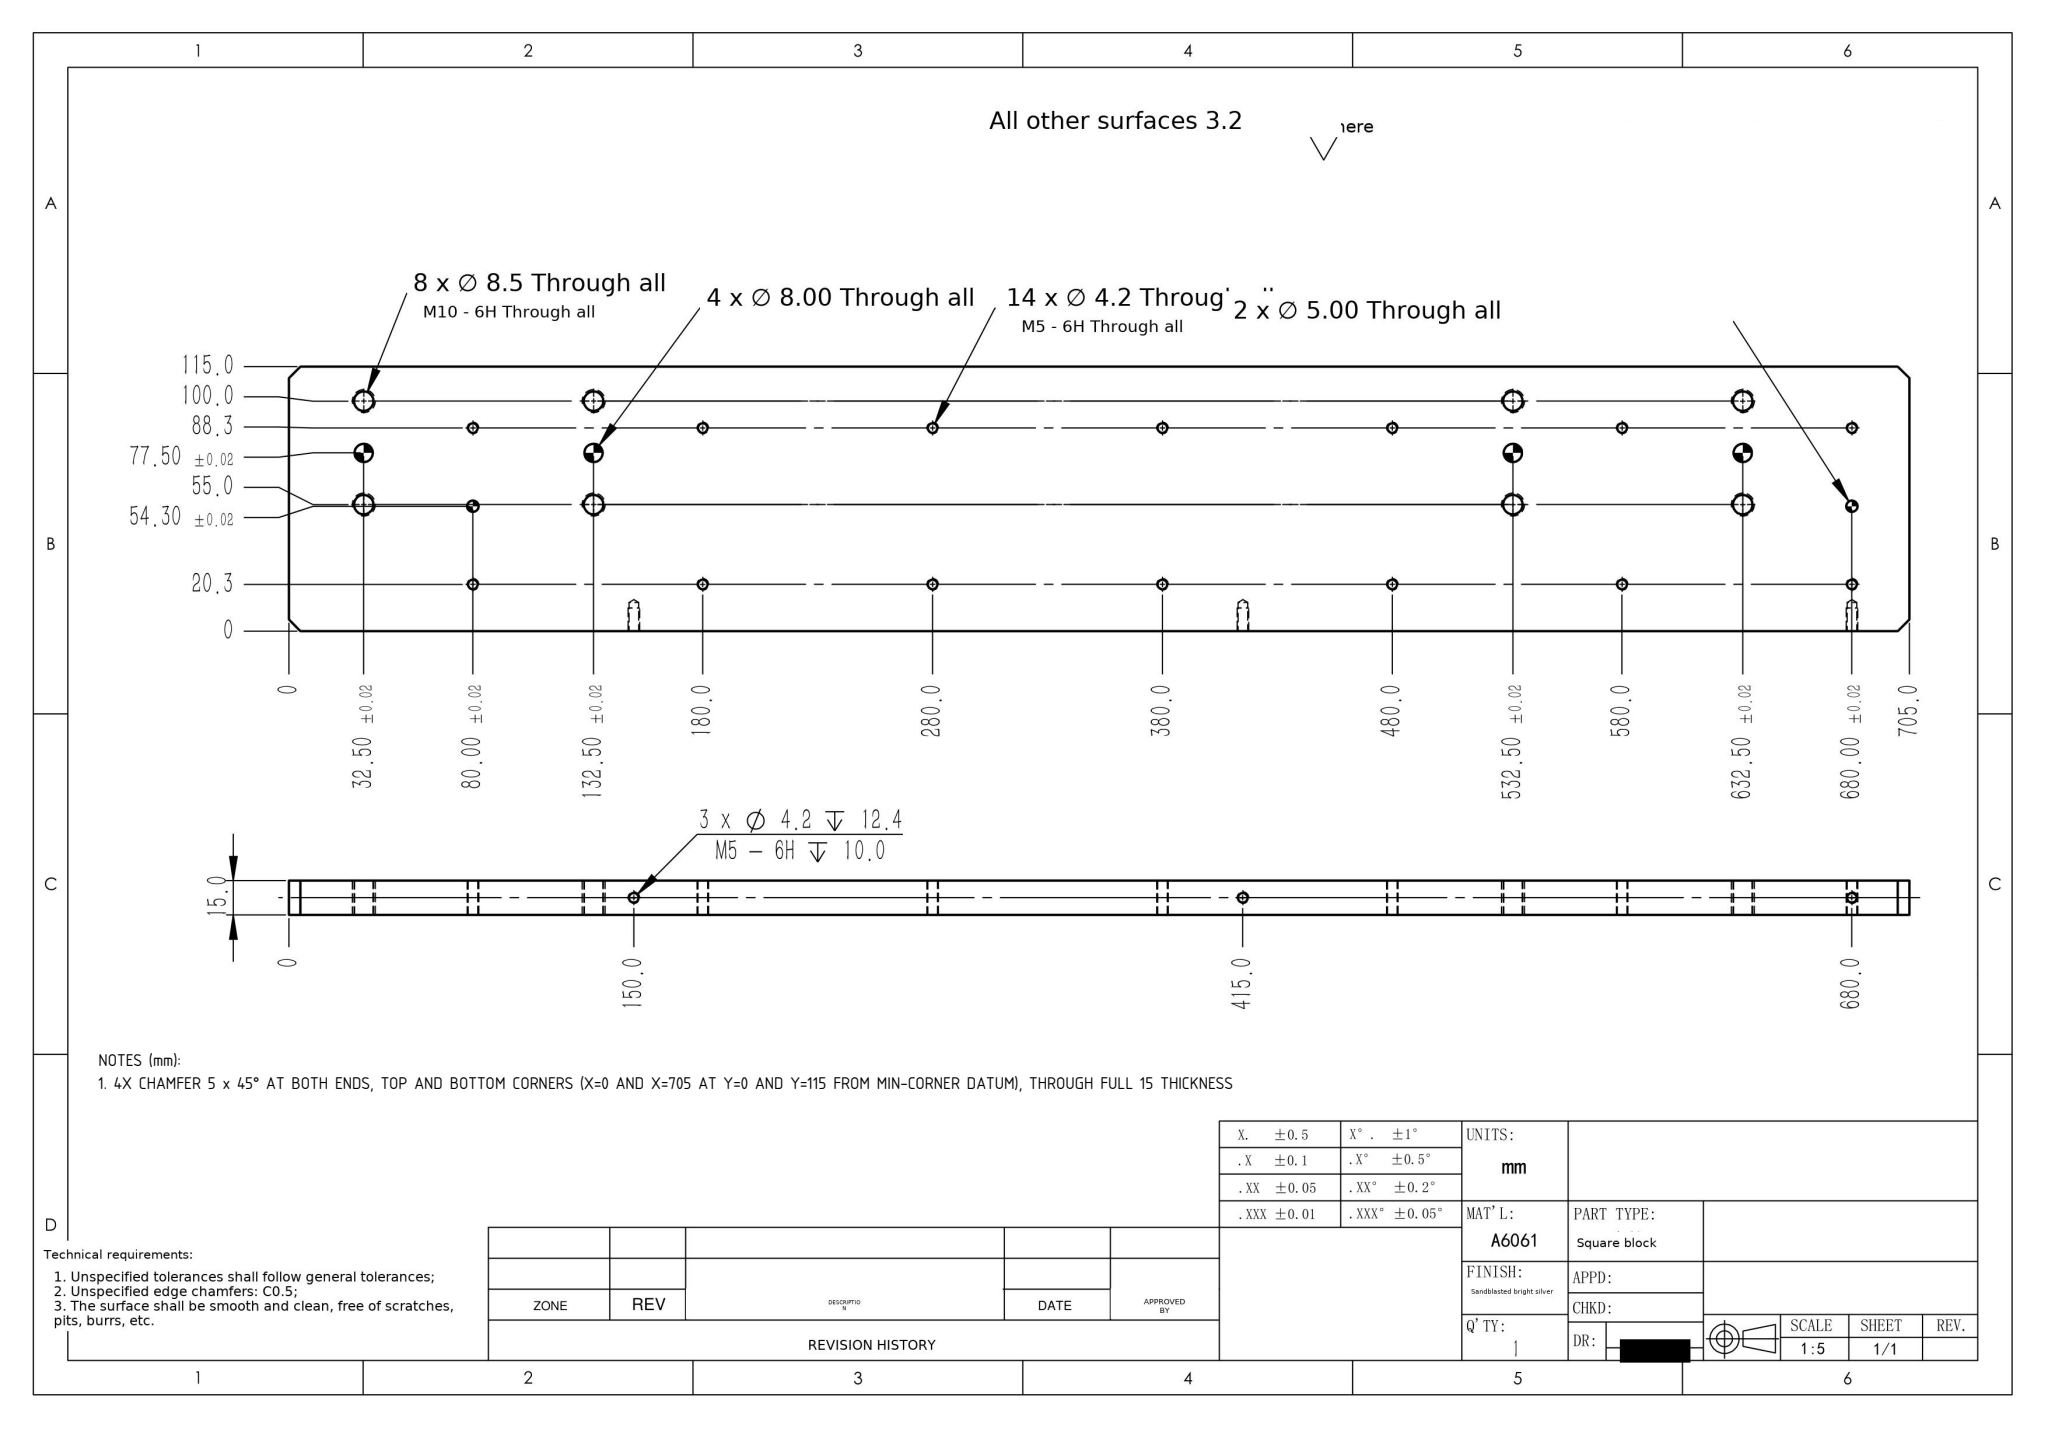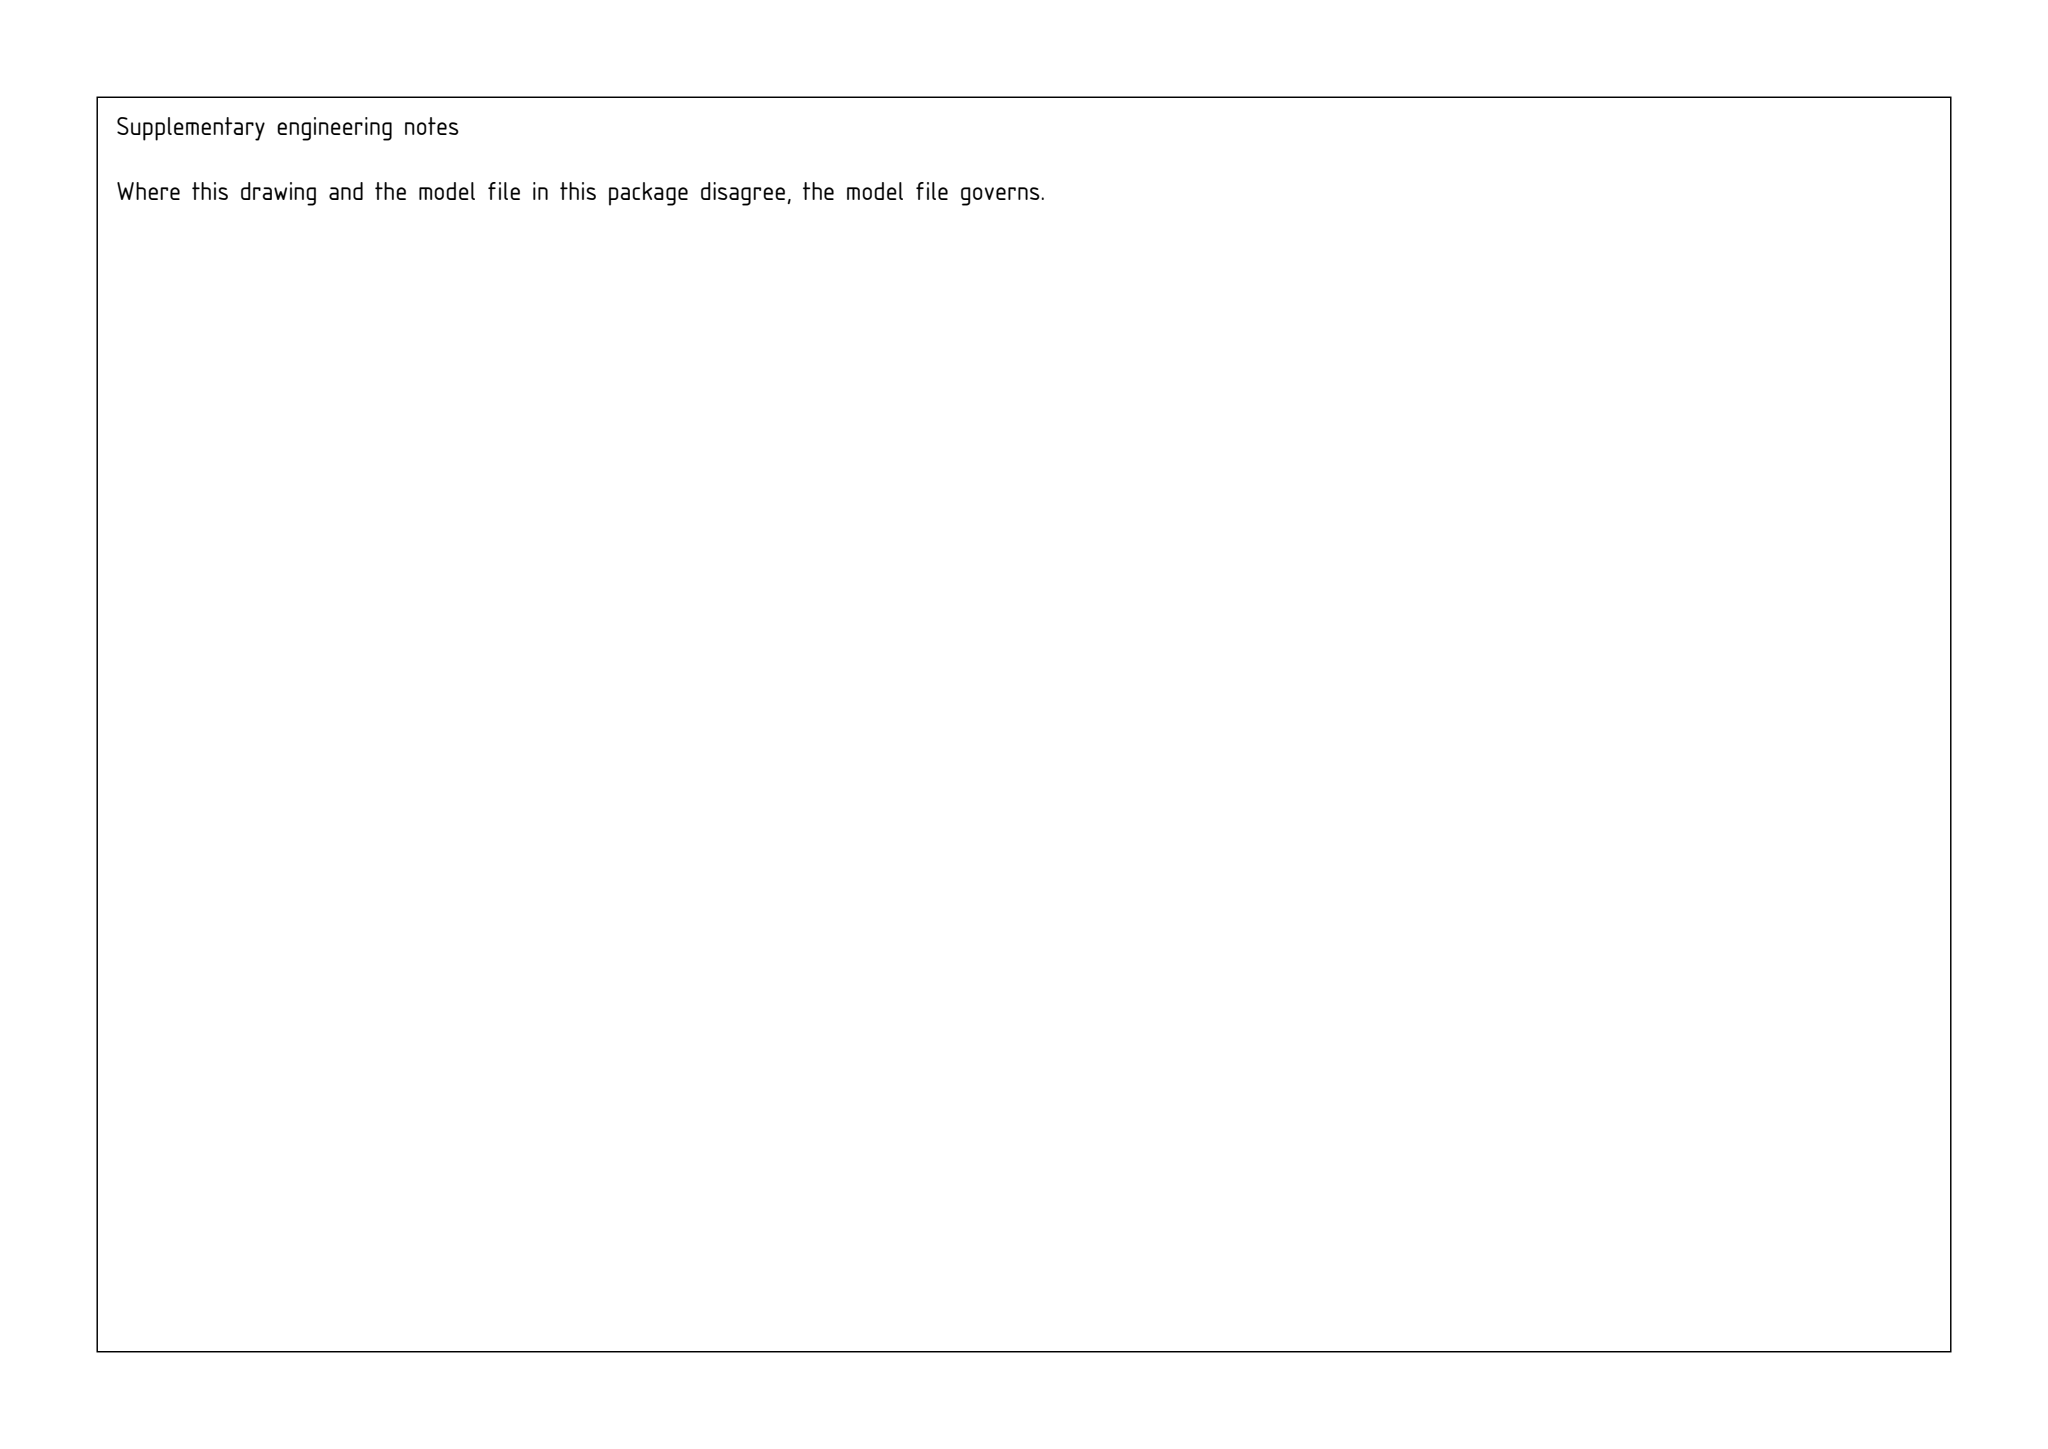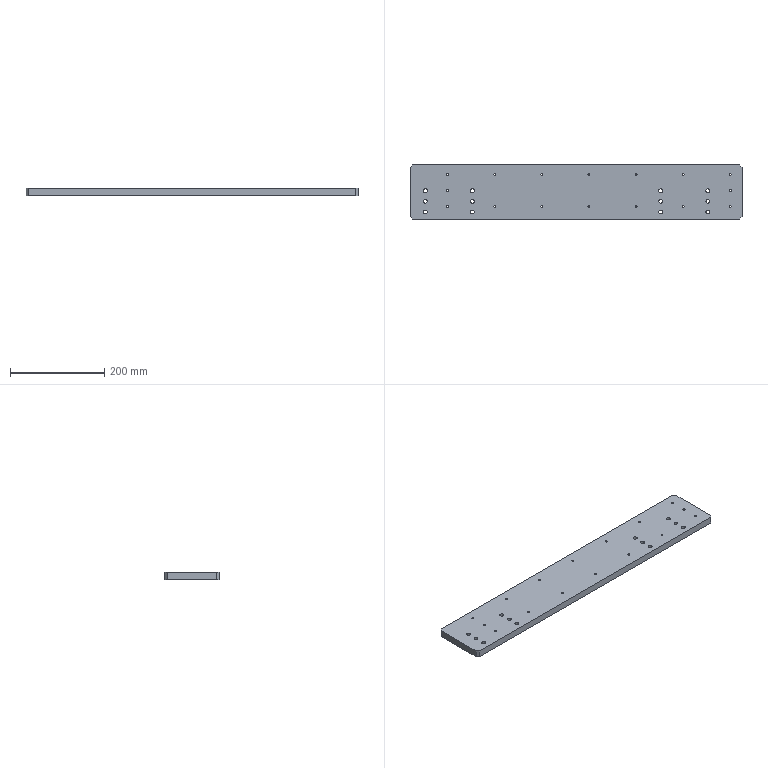Part | SolidWorks | mm | 1 solid | 78 faces | box 705 x 115 x 15 mm | volume 1201518 mm3 | cylinder 62 | plane 10 | cone 6 | commonest cylinder face diameters 4.2 x34 8.5 x16 8 x8 5 x4
Drawing notes:
4X CHAMFER 5 x 45° AT BOTH ENDS, TOP AND BOTTOM CORNERS (X=0 AND X=705 AT Y=0 AND Y=115 FROM MIN-CORNER DATUM), THROUGH FULL 15 THICKNESS | from the solid: inclined_planes: 4 faces at 45°/45°/90° to axes, size 5 x 5 x 15, bbox_from [0,0,0], [0,110,0], [700,0,0], [700,110,0]
build123d program:
from build123d import *

# Parameters (mm, degrees)
SKETCH1_W                  = 705
SKETCH1_H                  = 115
BOSS_EXTRUDE1_DEPTH        = 15
M5_TAPPED_HOLE1_D          = 4.2
LPATTERN1_COUNT            = 7
LPATTERN1_PITCH            = 100
SIZE_MM_DOWEL_PIN_HOLE_2_D = 5
M10_TAPPED_HOLE1_D         = 8.5
SIZE_MM_DOWEL_PIN_HOLE_0_D = 8
M5_TAPPED_HOLE2_D          = 4.2
M5_TAPPED_HOLE2_DEPTH      = 12.4
M5_TAPPED_HOLE2_TIP        = 1.262
LPATTERN2_COUNT            = 2
LPATTERN2_PITCH            = 500
CHAMFER1_SIZE              = 5


with BuildPart() as part:
    # Sketch1 → Boss-Extrude1 (new body)
    with BuildSketch(Plane.XY):
        Rectangle(SKETCH1_W, SKETCH1_H)
    extrude(amount=BOSS_EXTRUDE1_DEPTH)

    # M5 Tapped Hole1 (through all)
    with Locations(Plane.XY.offset(15)):
        with Locations((-272.5, 37.2), (-272.5, -30.8)):
            m5_tapped_hole1 = Hole(M5_TAPPED_HOLE1_D / 2)

    # LPattern1: M5 Tapped Hole1 ×7
    with Locations(*[(i * LPATTERN1_PITCH, 0, 0) for i in range(1, LPATTERN1_COUNT)]):
        add(m5_tapped_hole1, mode=Mode.SUBTRACT)

    # Size mm Dowel Pin Hole 2 (through all)
    with Locations(Plane(origin=(0, 0, 0), x_dir=(-1, 0, 0), z_dir=(0, 0, -1))):
        with Locations((-327.5, 3.2), (272.5, 3.2)):
            Hole(SIZE_MM_DOWEL_PIN_HOLE_2_D / 2)

    # M10 Tapped Hole1 (through all)
    with Locations(Plane.XY.offset(15)):
        with Locations((-320, 2.5), (-320, -42.5), (-220, -42.5), (-220, 2.5)):
            m10_tapped_hole1 = Hole(M10_TAPPED_HOLE1_D / 2)

    # Size mm Dowel Pin Hole 0 (through all)
    with Locations(Plane.XY.offset(15)):
        with Locations((-320, -20), (-220, -20)):
            size_mm_dowel_pin_hole_0 = Hole(SIZE_MM_DOWEL_PIN_HOLE_0_D / 2)

    # M5 Tapped Hole2
    with Locations(Plane(origin=(0, 57.5, 0), x_dir=(1, 0, 0), z_dir=(0, 1, 0))):
        with Locations((-202.5, -7.5), (62.5, -7.5), (327.5, -7.5)):
            Hole(M5_TAPPED_HOLE2_D / 2, depth=M5_TAPPED_HOLE2_DEPTH)
            with Locations((0, 0, -(M5_TAPPED_HOLE2_DEPTH + M5_TAPPED_HOLE2_TIP / 2))):  # 118° drill point
                Cone(0, M5_TAPPED_HOLE2_D / 2, M5_TAPPED_HOLE2_TIP, mode=Mode.SUBTRACT)

    # LPattern2: M10 Tapped Hole1, Size mm Dowel Pin Hole 0 ×2
    with Locations(*[(i * LPATTERN2_PITCH, 0, 0) for i in range(1, LPATTERN2_COUNT)]):
        add(m10_tapped_hole1, mode=Mode.SUBTRACT)
        add(size_mm_dowel_pin_hole_0, mode=Mode.SUBTRACT)

    # Chamfer1
    chamfer1_edges = [part.edges().sort_by_distance(p)[0] for p in [
        (352.5, -57.5, 7.5),
        (-352.5, -57.5, 7.5),
        (-352.5, 57.5, 7.5),
        (352.5, 57.5, 7.5),
    ]]
    chamfer(chamfer1_edges, length=CHAMFER1_SIZE)


solid = part.part